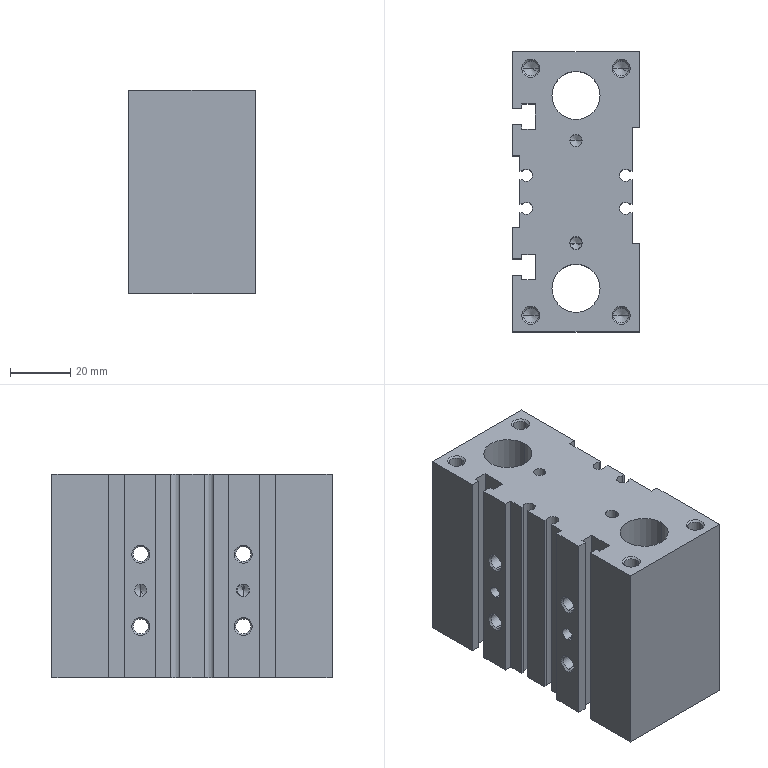Component | SolidWorks | MGPM25-30Z-M9P-1_MGPM25_30Z_0_BODY_2-1 | 1 solid | 176 faces | volume 189935 mm3 | cylinder 64 | plane 64 | cone 48 | commonest cylinder face diameters 4.917 x16 4 x12 9.5 x8 5.4 x8 8.566 x8 4.05 x4 16 x4 10 x2